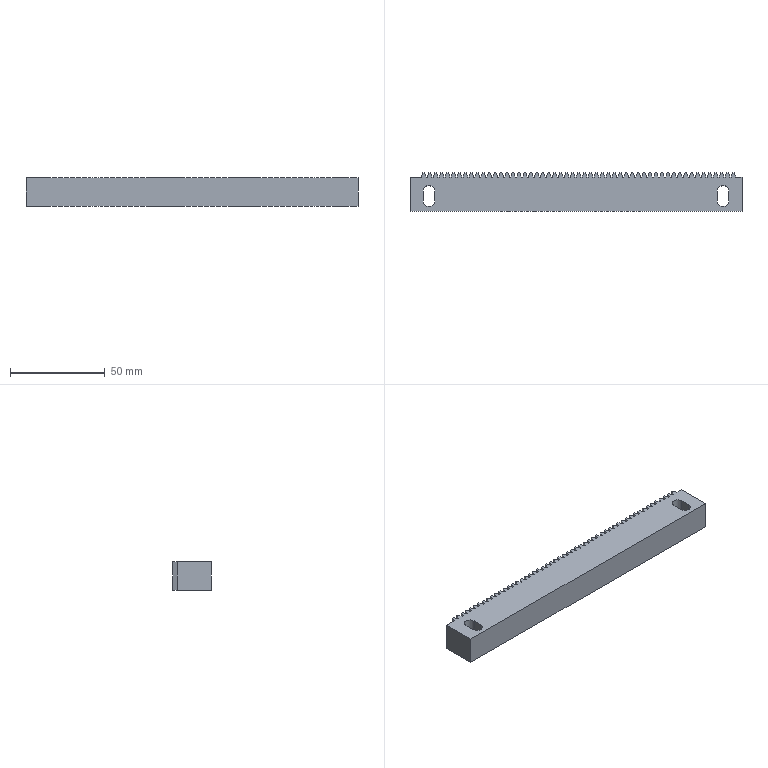Component | SolidWorks | Rack-2 | 1 solid | 226 faces | box 175 x 20.3 x 15 mm | volume 48464 mm3 | plane 222 | cylinder 4 | commonest cylinder face diameters 6 x4
build123d program:
from build123d import *

# Parameters (mm, degrees)
BOSS_EXTRUDE1_DEPTH = 15


with BuildPart() as part:
    # Sketch1 → Boss-Extrude1 (new body)
    with BuildSketch(Plane(origin=(0, 0, -7.5), x_dir=(-1, 0, 0), z_dir=(0, 0, -1))):
        Polygon((-83.4, 20.3), (-84.22, 18), (-87.5, 18), (-87.5, 0), (87.5, 0), (87.5, 18), (81.5, 18), (80.68, 20.3), (79.88, 20.3), (79.06, 18), (78.36, 18), (77.54, 20.3), (76.74, 20.3), (75.92, 18), (75.22, 18), (74.4, 20.3), (73.6, 20.3), (72.78, 18), (72.08, 18), (71.26, 20.3), (70.46, 20.3), (69.64, 18), (68.94, 18), (68.12, 20.3), (67.32, 20.3), (66.5, 18), (65.8, 18), (64.98, 20.3), (64.18, 20.3), (63.36, 18), (62.66, 18), (61.84, 20.3), (61.04, 20.3), (60.22, 18), (59.52, 18), (58.7, 20.3), (57.9, 20.3), (57.08, 18), (56.38, 18), (55.56, 20.3), (54.76, 20.3), (53.94, 18), (53.24, 18), (52.42, 20.3), (51.62, 20.3), (50.8, 18), (50.1, 18), (49.28, 20.3), (48.48, 20.3), (47.66, 18), (46.96, 18), (46.14, 20.3), (45.34, 20.3), (44.52, 18), (43.82, 18), (43, 20.3), (42.2, 20.3), (41.38, 18), (40.68, 18), (39.86, 20.3), (39.06, 20.3), (38.24, 18), (37.54, 18), (36.72, 20.3), (35.92, 20.3), (35.1, 18), (34.4, 18), (33.58, 20.3), (32.78, 20.3), (31.96, 18), (31.26, 18), (30.44, 20.3), (29.64, 20.3), (28.82, 18), (28.12, 18), (27.3, 20.3), (26.5, 20.3), (25.68, 18), (24.98, 18), (24.16, 20.3), (23.36, 20.3), (22.54, 18), (21.84, 18), (21.02, 20.3), (20.22, 20.3), (19.4, 18), (18.7, 18), (17.88, 20.3), (17.08, 20.3), (16.26, 18), (15.56, 18), (14.74, 20.3), (13.94, 20.3), (13.12, 18), (12.42, 18), (11.6, 20.3), (10.8, 20.3), (9.98, 18), (9.28, 18), (8.46, 20.3), (7.66, 20.3), (6.84, 18), (6.14, 18), (5.32, 20.3), (4.52, 20.3), (3.7, 18), (3, 18), (2.18, 20.3), (1.38, 20.3), (0.56, 18), (-0.14, 18), (-0.96, 20.3), (-1.76, 20.3), (-2.58, 18), (-3.28, 18), (-4.1, 20.3), (-4.9, 20.3), (-5.72, 18), (-6.42, 18), (-7.24, 20.3), (-8.04, 20.3), (-8.86, 18), (-9.56, 18), (-10.38, 20.3), (-11.18, 20.3), (-12, 18), (-12.7, 18), (-13.52, 20.3), (-14.32, 20.3), (-15.14, 18), (-15.84, 18), (-16.66, 20.3), (-17.46, 20.3), (-18.28, 18), (-18.98, 18), (-19.8, 20.3), (-20.6, 20.3), (-21.42, 18), (-22.12, 18), (-22.94, 20.3), (-23.74, 20.3), (-24.56, 18), (-25.26, 18), (-26.08, 20.3), (-26.88, 20.3), (-27.7, 18), (-28.4, 18), (-29.22, 20.3), (-30.02, 20.3), (-30.84, 18), (-31.54, 18), (-32.36, 20.3), (-33.16, 20.3), (-33.98, 18), (-34.68, 18), (-35.5, 20.3), (-36.3, 20.3), (-37.12, 18), (-37.82, 18), (-38.64, 20.3), (-39.44, 20.3), (-40.26, 18), (-40.96, 18), (-41.78, 20.3), (-42.58, 20.3), (-43.4, 18), (-44.1, 18), (-44.92, 20.3), (-45.72, 20.3), (-46.54, 18), (-47.24, 18), (-48.06, 20.3), (-48.86, 20.3), (-49.68, 18), (-50.38, 18), (-51.2, 20.3), (-52, 20.3), (-52.82, 18), (-53.52, 18), (-54.34, 20.3), (-55.14, 20.3), (-55.96, 18), (-56.66, 18), (-57.48, 20.3), (-58.28, 20.3), (-59.1, 18), (-59.8, 18), (-60.62, 20.3), (-61.42, 20.3), (-62.24, 18), (-62.94, 18), (-63.76, 20.3), (-64.56, 20.3), (-65.38, 18), (-66.08, 18), (-66.9, 20.3), (-67.7, 20.3), (-68.52, 18), (-69.22, 18), (-70.04, 20.3), (-70.84, 20.3), (-71.66, 18), (-72.36, 18), (-73.18, 20.3), (-73.98, 20.3), (-74.8, 18), (-75.5, 18), (-76.32, 20.3), (-77.12, 20.3), (-77.94, 18), (-78.64, 18), (-79.46, 20.3), (-80.26, 20.3), (-81.08, 18), (-81.78, 18), (-82.6, 20.3), align=None)
        with BuildLine():
            Line((74.5, 5.5), (74.5, 10.5))
            ThreePointArc((74.5, 10.5), (77.5, 13.5), (80.5, 10.5))
            Line((80.5, 10.5), (80.5, 5.5))
            ThreePointArc((80.5, 5.5), (77.5, 2.5), (74.5, 5.5))
        make_face(mode=Mode.SUBTRACT)
        with BuildLine():
            Line((-80.5, 5.5), (-80.5, 10.5))
            ThreePointArc((-80.5, 10.5), (-77.5, 13.5), (-74.5, 10.5))
            Line((-74.5, 10.5), (-74.5, 5.5))
            ThreePointArc((-74.5, 5.5), (-77.5, 2.5), (-80.5, 5.5))
        make_face(mode=Mode.SUBTRACT)
    extrude(amount=-BOSS_EXTRUDE1_DEPTH)


solid = part.part

# Placed as in the assembly
solid = solid.moved(Location((-257.5, 531.68, 255), (0, 0, 0)))